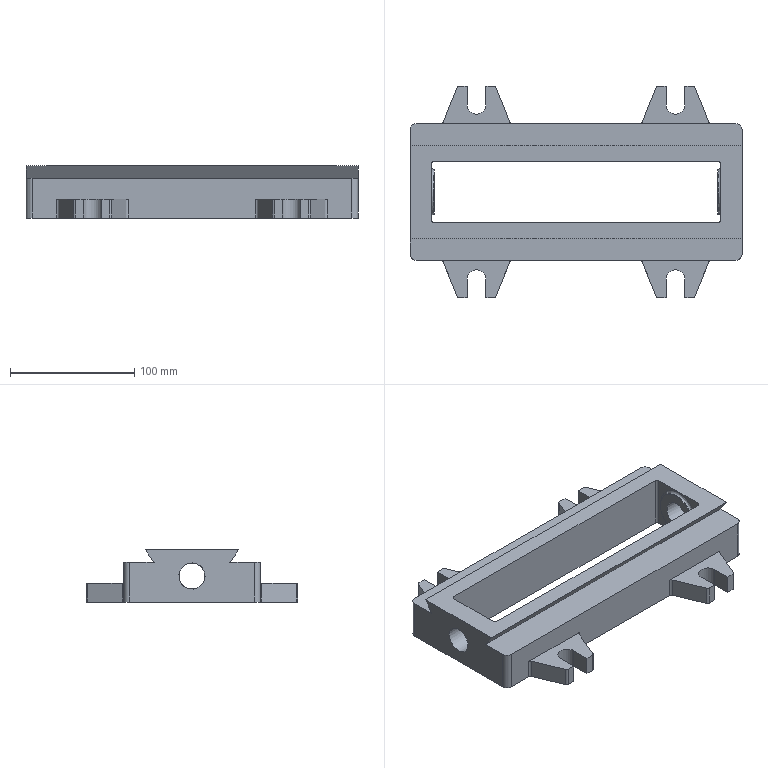Component | NX | BASE | 1 solid | 78 faces | volume 690684 mm3 | plane 44 | cylinder 32 | torus 2 | commonest cylinder face diameters 4 x20 10 x4 15 x4 21 x2 36 x2